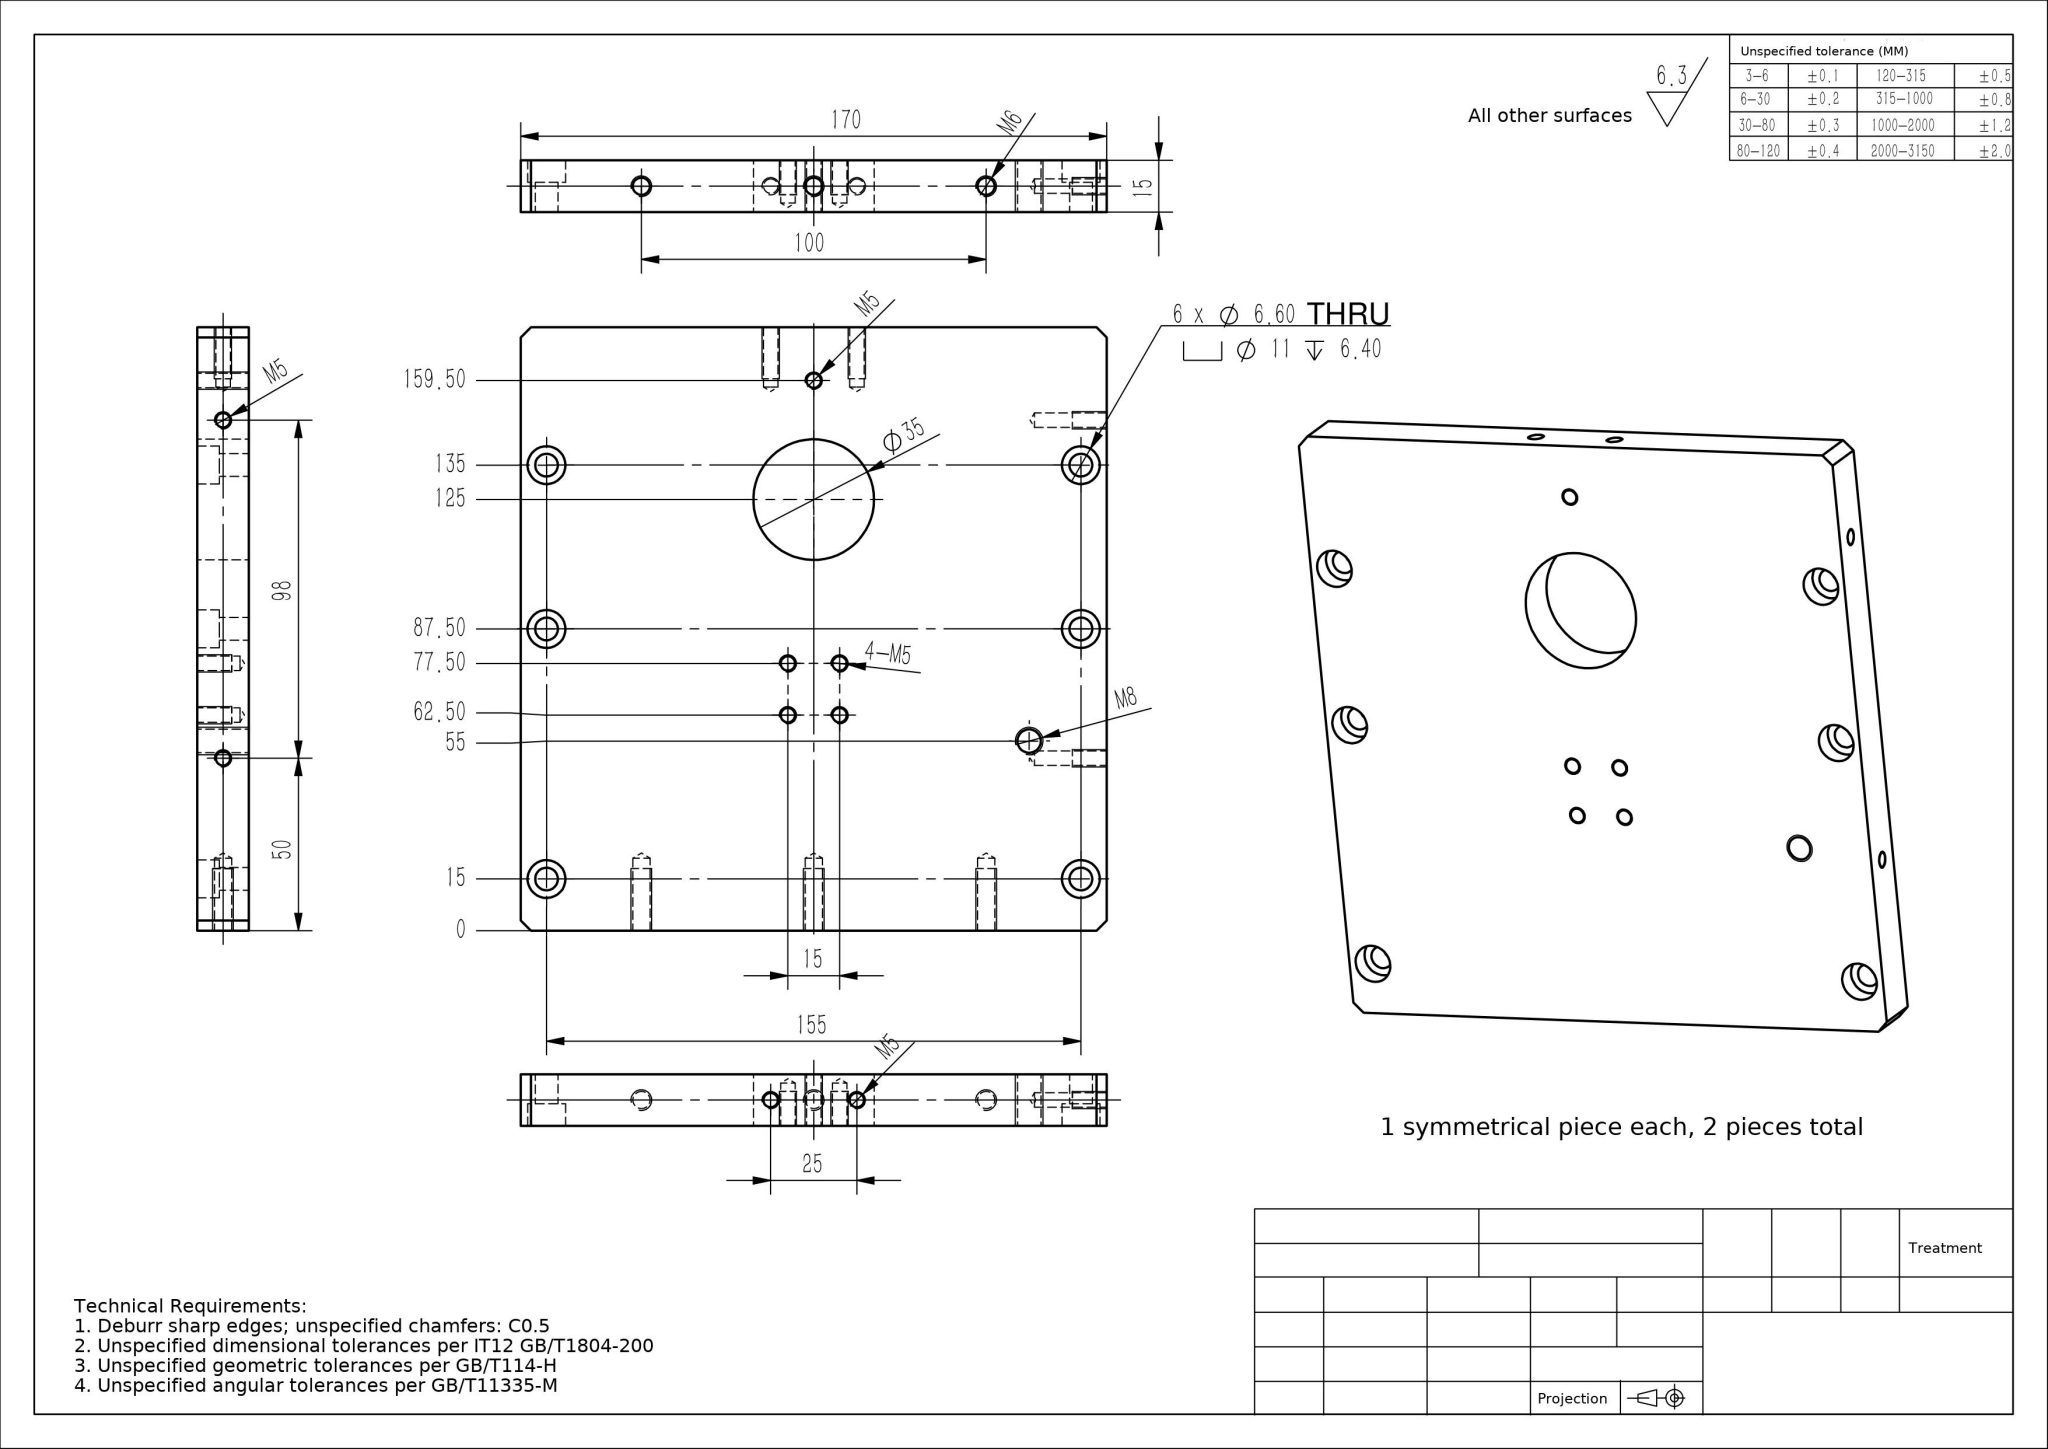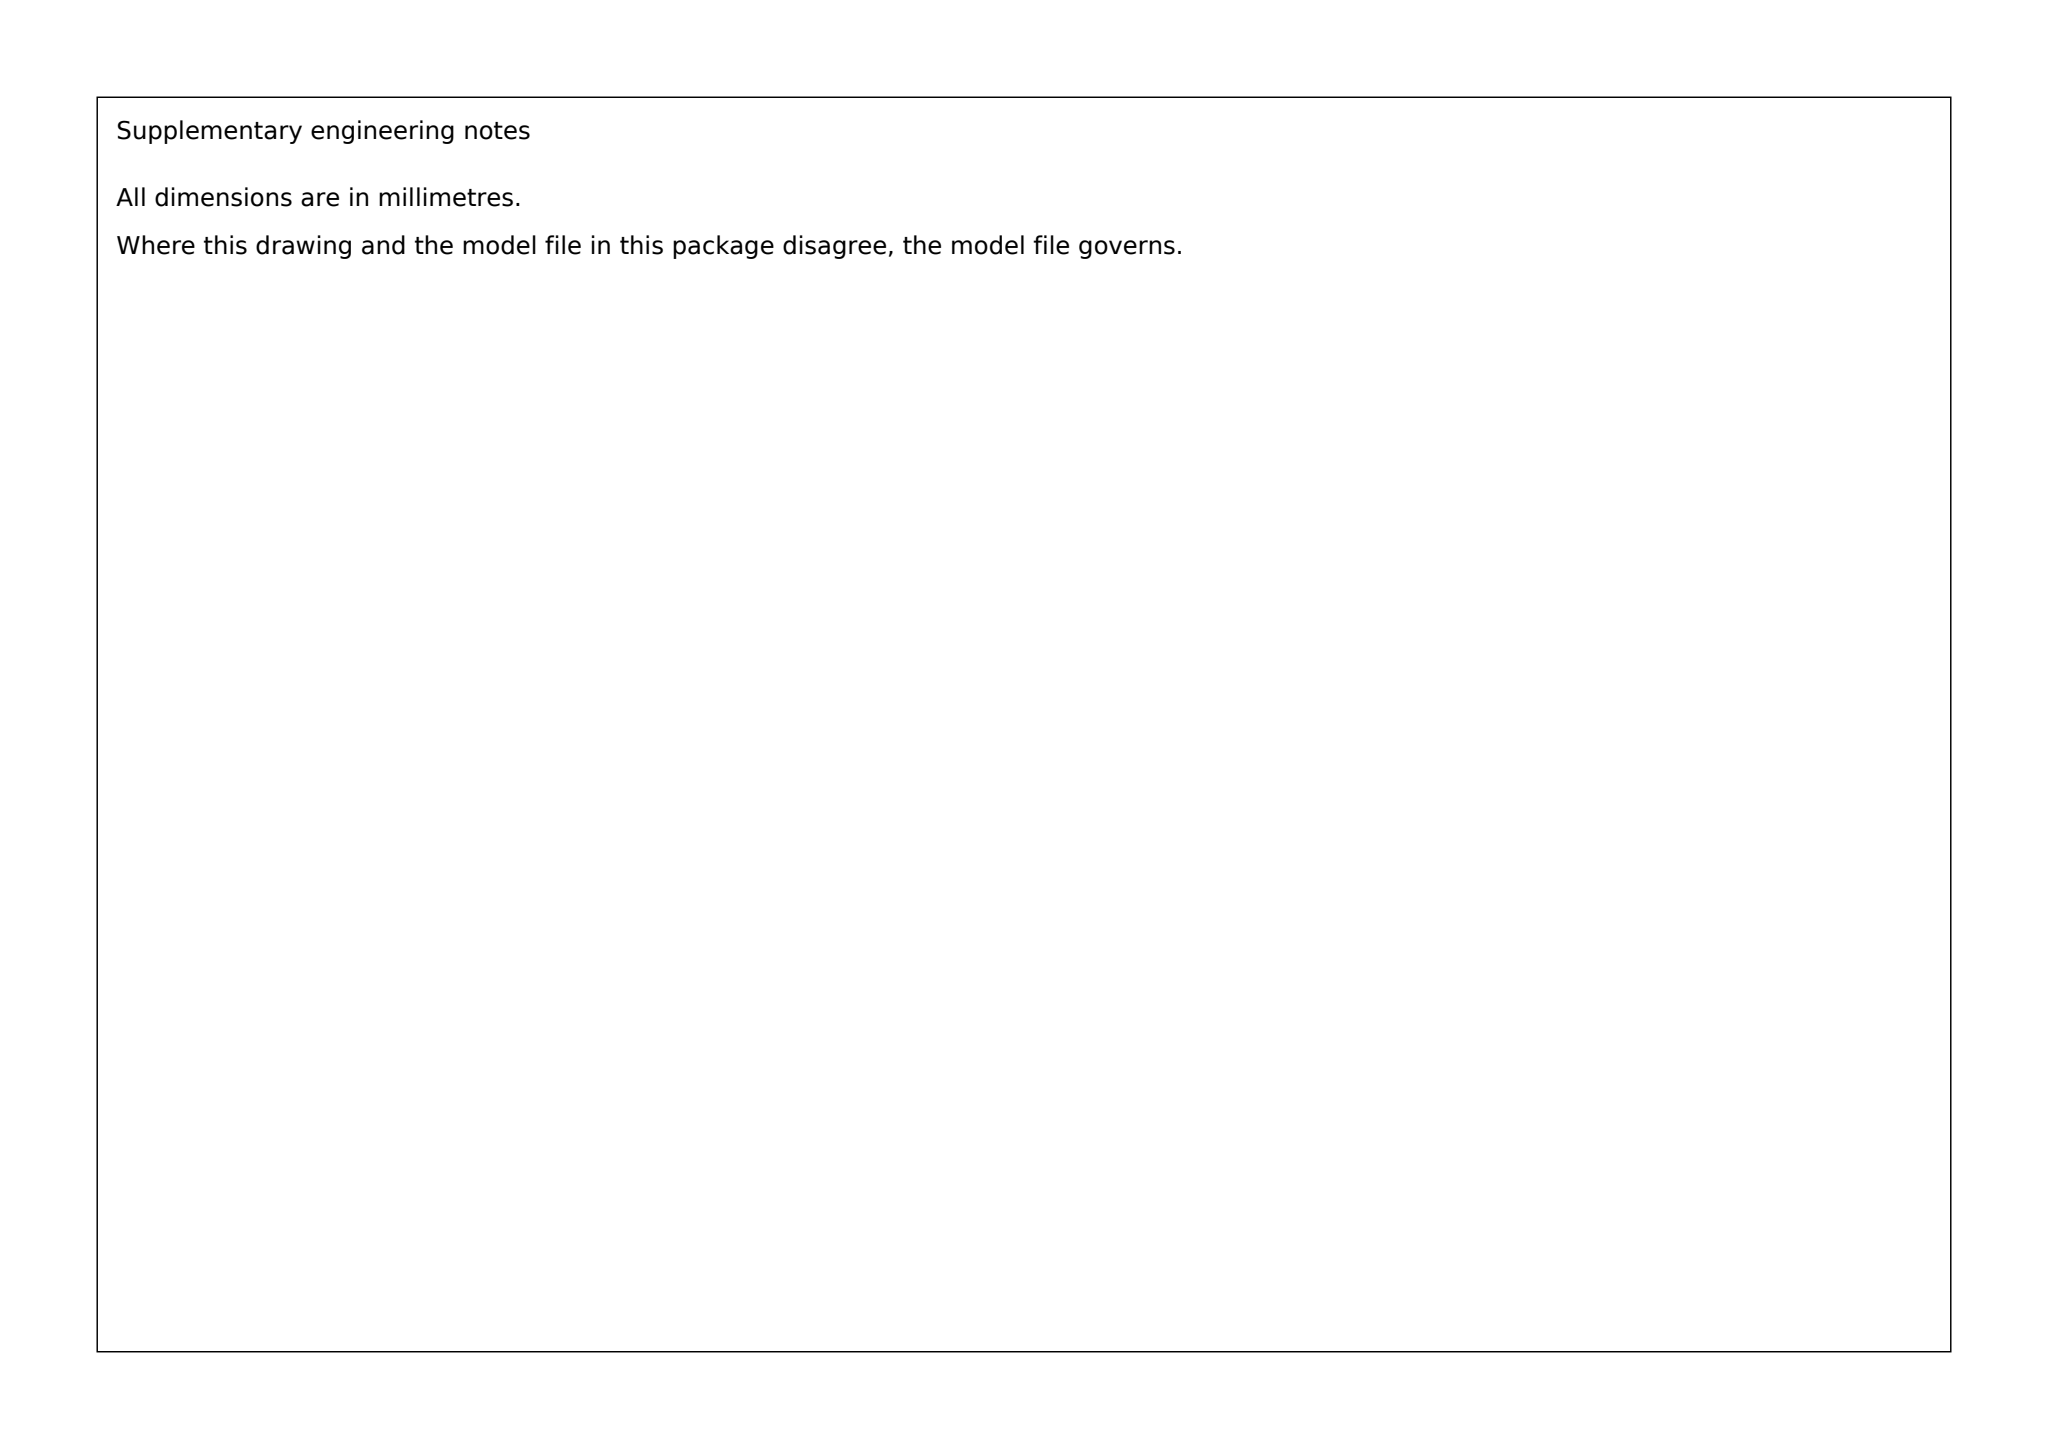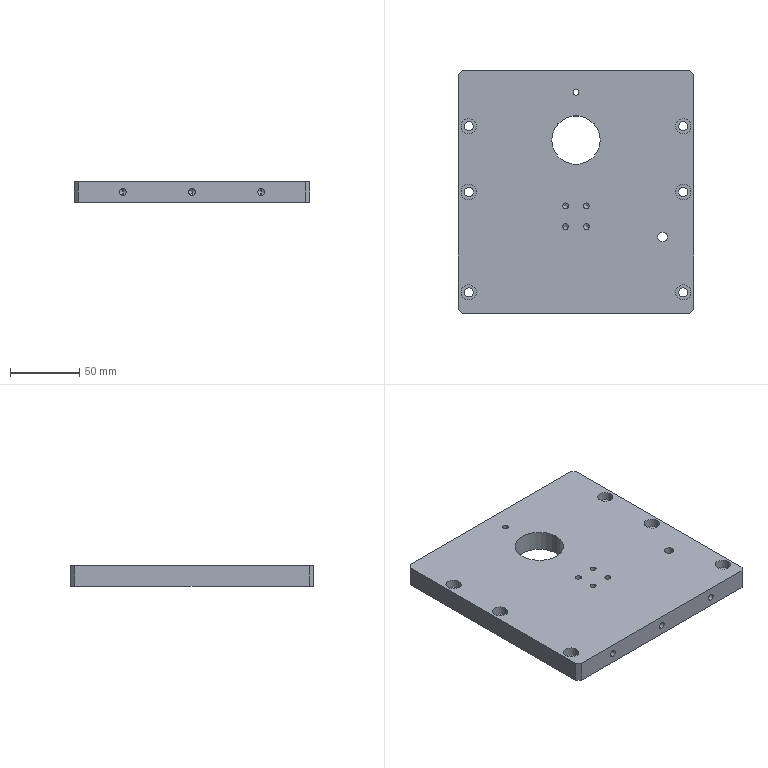Part | SolidWorks | mm | 1 solid | 90 faces | box 170 x 175 x 15 mm | volume 422317 mm3 | cylinder 52 | cone 22 | plane 16 | commonest cylinder face diameters 4.2 x18 11 x12 6.6 x12 5 x6 35 x2 6.8 x2
build123d program:
from build123d import *

# Parameters (mm, degrees)
SKETCH1_W                                       = 170
SKETCH1_H                                       = 175
BOSS_EXTRUDE1_DEPTH                             = 15
M6_HEX_SOCKET_HEAD_CAP_SCREW_CBORE2_D           = 6.6
M6_HEX_SOCKET_HEAD_CAP_SCREW_CBORE2_CBORE_D     = 11
M6_HEX_SOCKET_HEAD_CAP_SCREW_CBORE2_CBORE_DEPTH = 6.4
CHAMFER1_SIZE                                   = 3
M8_TAPPED_HOLE1_D                               = 6.8
M8_TAPPED_HOLE1_DEPTH                           = 19.75
M8_TAPPED_HOLE1_TIP                             = 2.043
M5_TAPPED_HOLE1_D                               = 4.2
M5_TAPPED_HOLE1_DEPTH                           = 17.4
M5_TAPPED_HOLE1_TIP                             = 1.262
M6_TAPPED_HOLE1_D                               = 5
M6_TAPPED_HOLE1_DEPTH                           = 21
M6_TAPPED_HOLE1_TIP                             = 1.502
M5_TAPPED_HOLE4_D                               = 4.2
M5_TAPPED_HOLE4_DEPTH                           = 12.4
M5_TAPPED_HOLE4_TIP                             = 1.262
SKETCH23_R                                      = 17.5
CUT_EXTRUDE1_DEPTH                              = 30
M5_TAPPED_HOLE5_D                               = 4.2
M5_TAPPED_HOLE6_D                               = 4.2
M5_TAPPED_HOLE6_DEPTH                           = 21
M5_TAPPED_HOLE6_TIP                             = 1.262


with BuildPart() as part:
    # Sketch1 → Boss-Extrude1 (new body)
    with BuildSketch(Plane.XY):
        Rectangle(SKETCH1_W, SKETCH1_H)
    extrude(amount=BOSS_EXTRUDE1_DEPTH)

    # M6 Hex Socket Head Cap Screw CBORE2 (through all)
    with Locations(Plane.XY.offset(15)):
        with Locations((-77.5, 47.5), (-77.5, 0), (-77.5, -72.5), (77.5, -72.5), (77.5, 0), (77.5, 47.5)):
            CounterBoreHole(M6_HEX_SOCKET_HEAD_CAP_SCREW_CBORE2_D / 2, M6_HEX_SOCKET_HEAD_CAP_SCREW_CBORE2_CBORE_D / 2, M6_HEX_SOCKET_HEAD_CAP_SCREW_CBORE2_CBORE_DEPTH)

    # Chamfer1
    chamfer1_edges = [part.edges().sort_by_distance(p)[0] for p in [
        (85, -87.5, 7.5),
        (-85, -87.5, 7.5),
        (-85, 87.5, 7.5),
        (85, 87.5, 7.5),
    ]]
    chamfer(chamfer1_edges, length=CHAMFER1_SIZE)

    # M8 Tapped Hole1
    with Locations(Plane.XY.offset(15)):
        with Locations((62.5, -32.5)):
            Hole(M8_TAPPED_HOLE1_D / 2, depth=M8_TAPPED_HOLE1_DEPTH)
            with Locations((0, 0, -(M8_TAPPED_HOLE1_DEPTH + M8_TAPPED_HOLE1_TIP / 2))):  # 118° drill point
                Cone(0, M8_TAPPED_HOLE1_D / 2, M8_TAPPED_HOLE1_TIP, mode=Mode.SUBTRACT)

    # M5 Tapped Hole1
    with Locations(Plane(origin=(0, 87.5, 0), x_dir=(1, 0, 0), z_dir=(0, 1, 0))):
        with Locations((12.5, -7.5), (-12.5, -7.5)):
            Hole(M5_TAPPED_HOLE1_D / 2, depth=M5_TAPPED_HOLE1_DEPTH)
            with Locations((0, 0, -(M5_TAPPED_HOLE1_DEPTH + M5_TAPPED_HOLE1_TIP / 2))):  # 118° drill point
                Cone(0, M5_TAPPED_HOLE1_D / 2, M5_TAPPED_HOLE1_TIP, mode=Mode.SUBTRACT)

    # M6 Tapped Hole1
    with Locations(Plane(origin=(0, -87.5, 0), x_dir=(-1, 0, 0), z_dir=(0, -1, 0))):
        with Locations((0, -7.5), (-50, -7.5), (50, -7.5)):
            Hole(M6_TAPPED_HOLE1_D / 2, depth=M6_TAPPED_HOLE1_DEPTH)
            with Locations((0, 0, -(M6_TAPPED_HOLE1_DEPTH + M6_TAPPED_HOLE1_TIP / 2))):  # 118° drill point
                Cone(0, M6_TAPPED_HOLE1_D / 2, M6_TAPPED_HOLE1_TIP, mode=Mode.SUBTRACT)

    # M5 Tapped Hole4
    with Locations(Plane.XY.offset(15)):
        with Locations((7.5, -10), (-7.5, -10), (-7.5, -25), (7.5, -25)):
            Hole(M5_TAPPED_HOLE4_D / 2, depth=M5_TAPPED_HOLE4_DEPTH)
            with Locations((0, 0, -(M5_TAPPED_HOLE4_DEPTH + M5_TAPPED_HOLE4_TIP / 2))):  # 118° drill point
                Cone(0, M5_TAPPED_HOLE4_D / 2, M5_TAPPED_HOLE4_TIP, mode=Mode.SUBTRACT)

    # Sketch23 → Cut-Extrude1 (cut)
    with BuildSketch(Plane.XY.offset(15)):
        with Locations((0, 37.5)):
            Circle(SKETCH23_R)
    extrude(amount=-CUT_EXTRUDE1_DEPTH, mode=Mode.SUBTRACT)

    # M5 Tapped Hole5 (through all)
    with Locations(Plane.XY.offset(15)):
        with Locations((0, 72)):
            Hole(M5_TAPPED_HOLE5_D / 2)

    # M5 Tapped Hole6
    with Locations(Plane(origin=(85, 0, 0), x_dir=(0, 0, -1), z_dir=(1, 0, 0))):
        with Locations((-7.5, 60.5), (-7.5, -37.5)):
            Hole(M5_TAPPED_HOLE6_D / 2, depth=M5_TAPPED_HOLE6_DEPTH)
            with Locations((0, 0, -(M5_TAPPED_HOLE6_DEPTH + M5_TAPPED_HOLE6_TIP / 2))):  # 118° drill point
                Cone(0, M5_TAPPED_HOLE6_D / 2, M5_TAPPED_HOLE6_TIP, mode=Mode.SUBTRACT)


solid = part.part